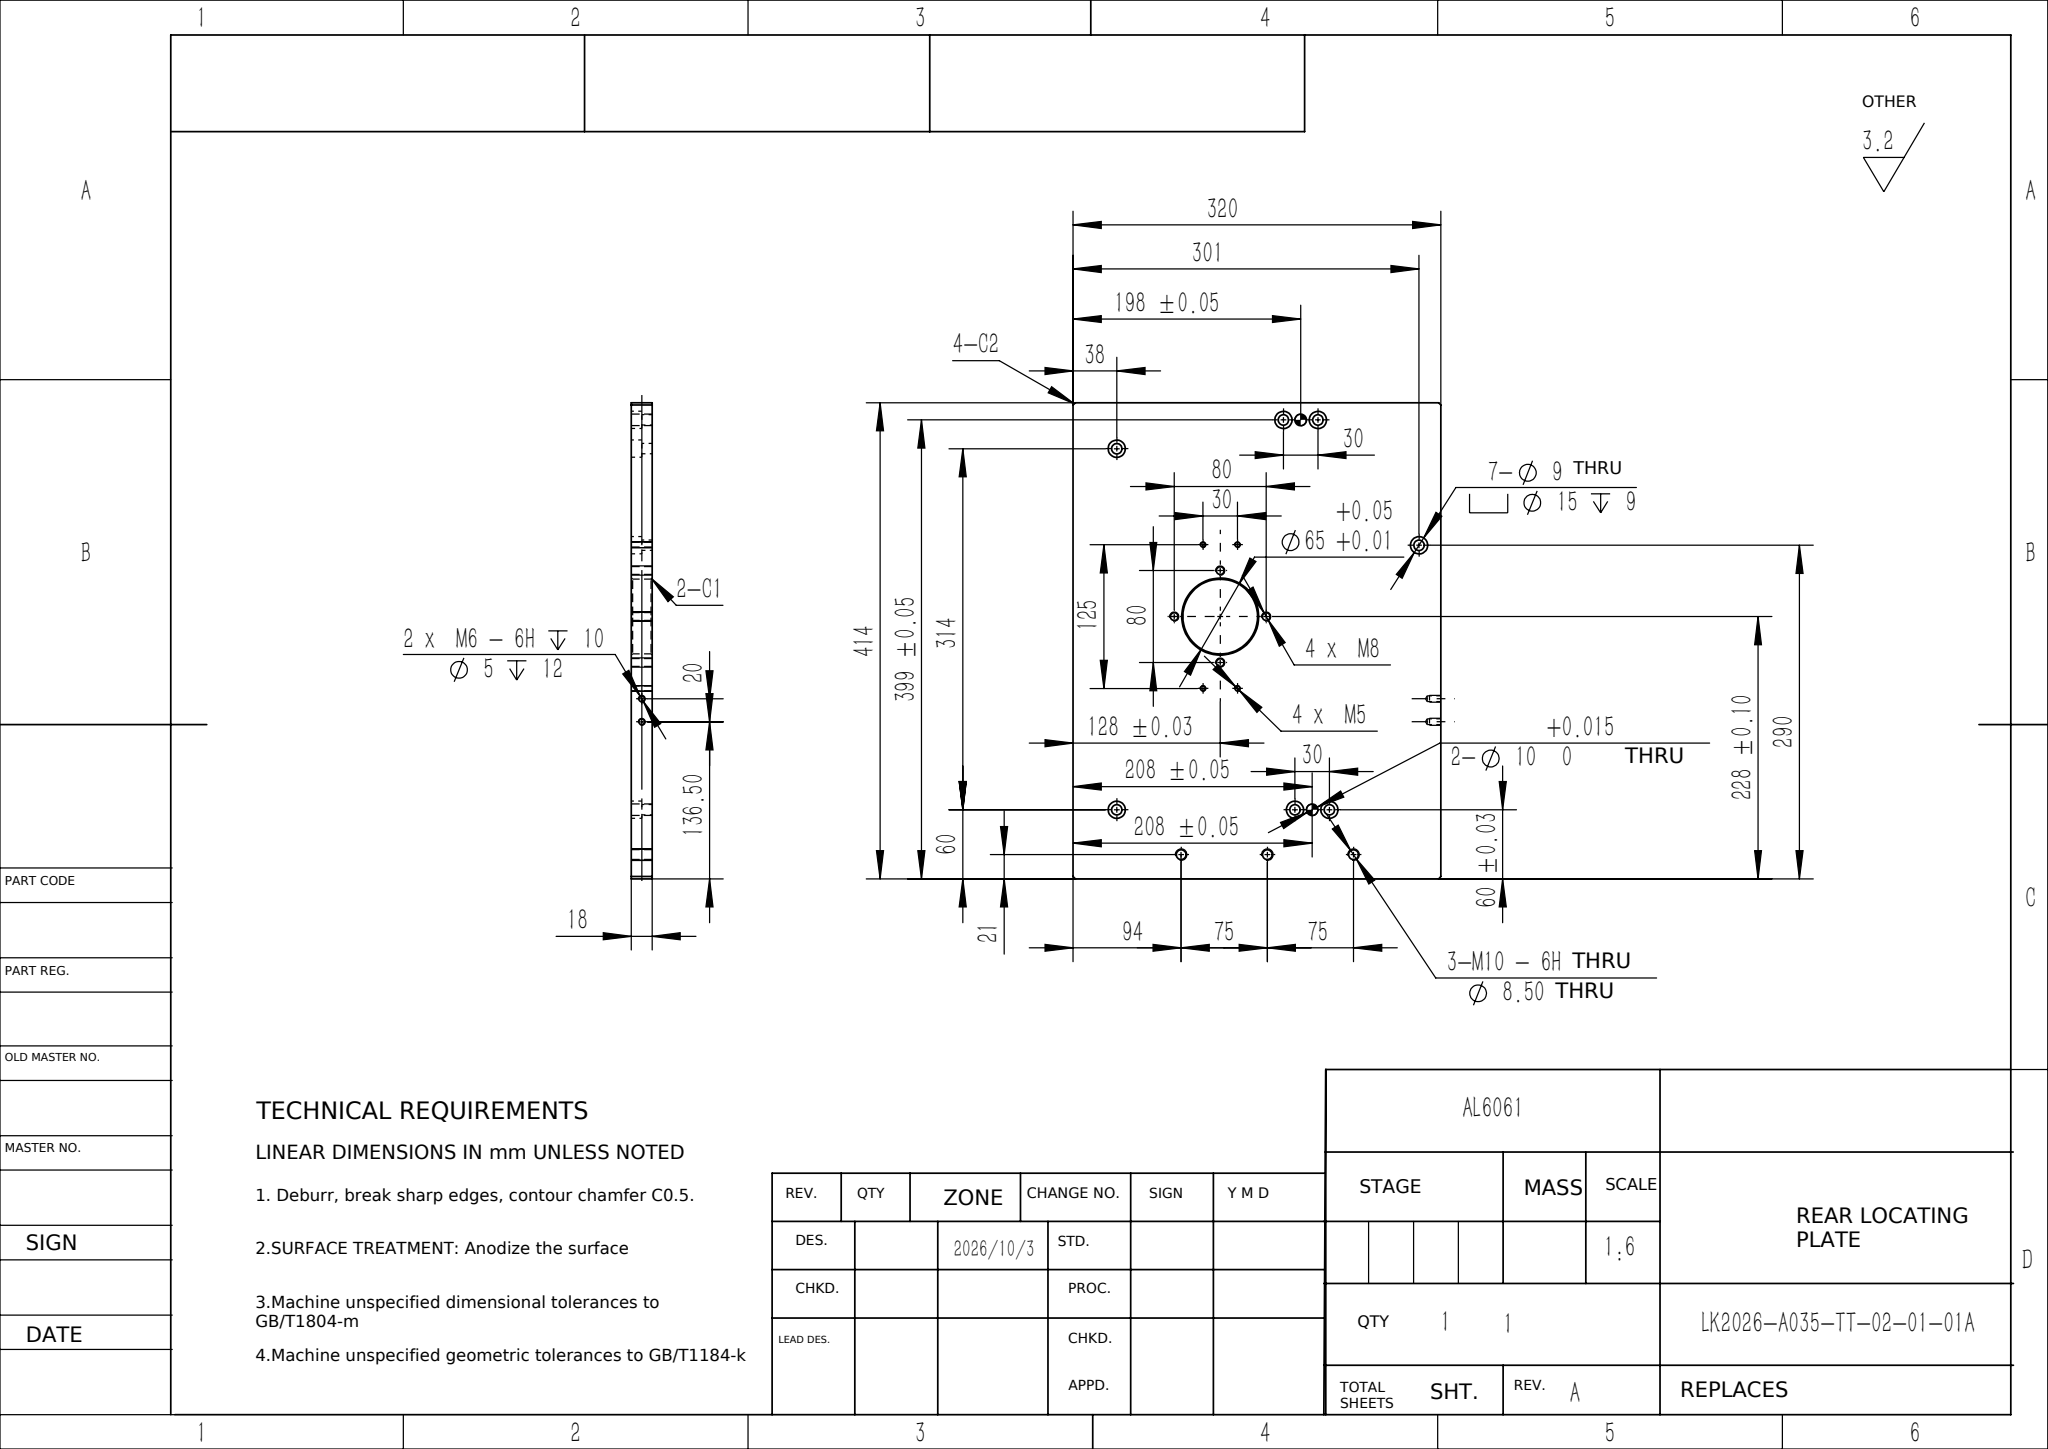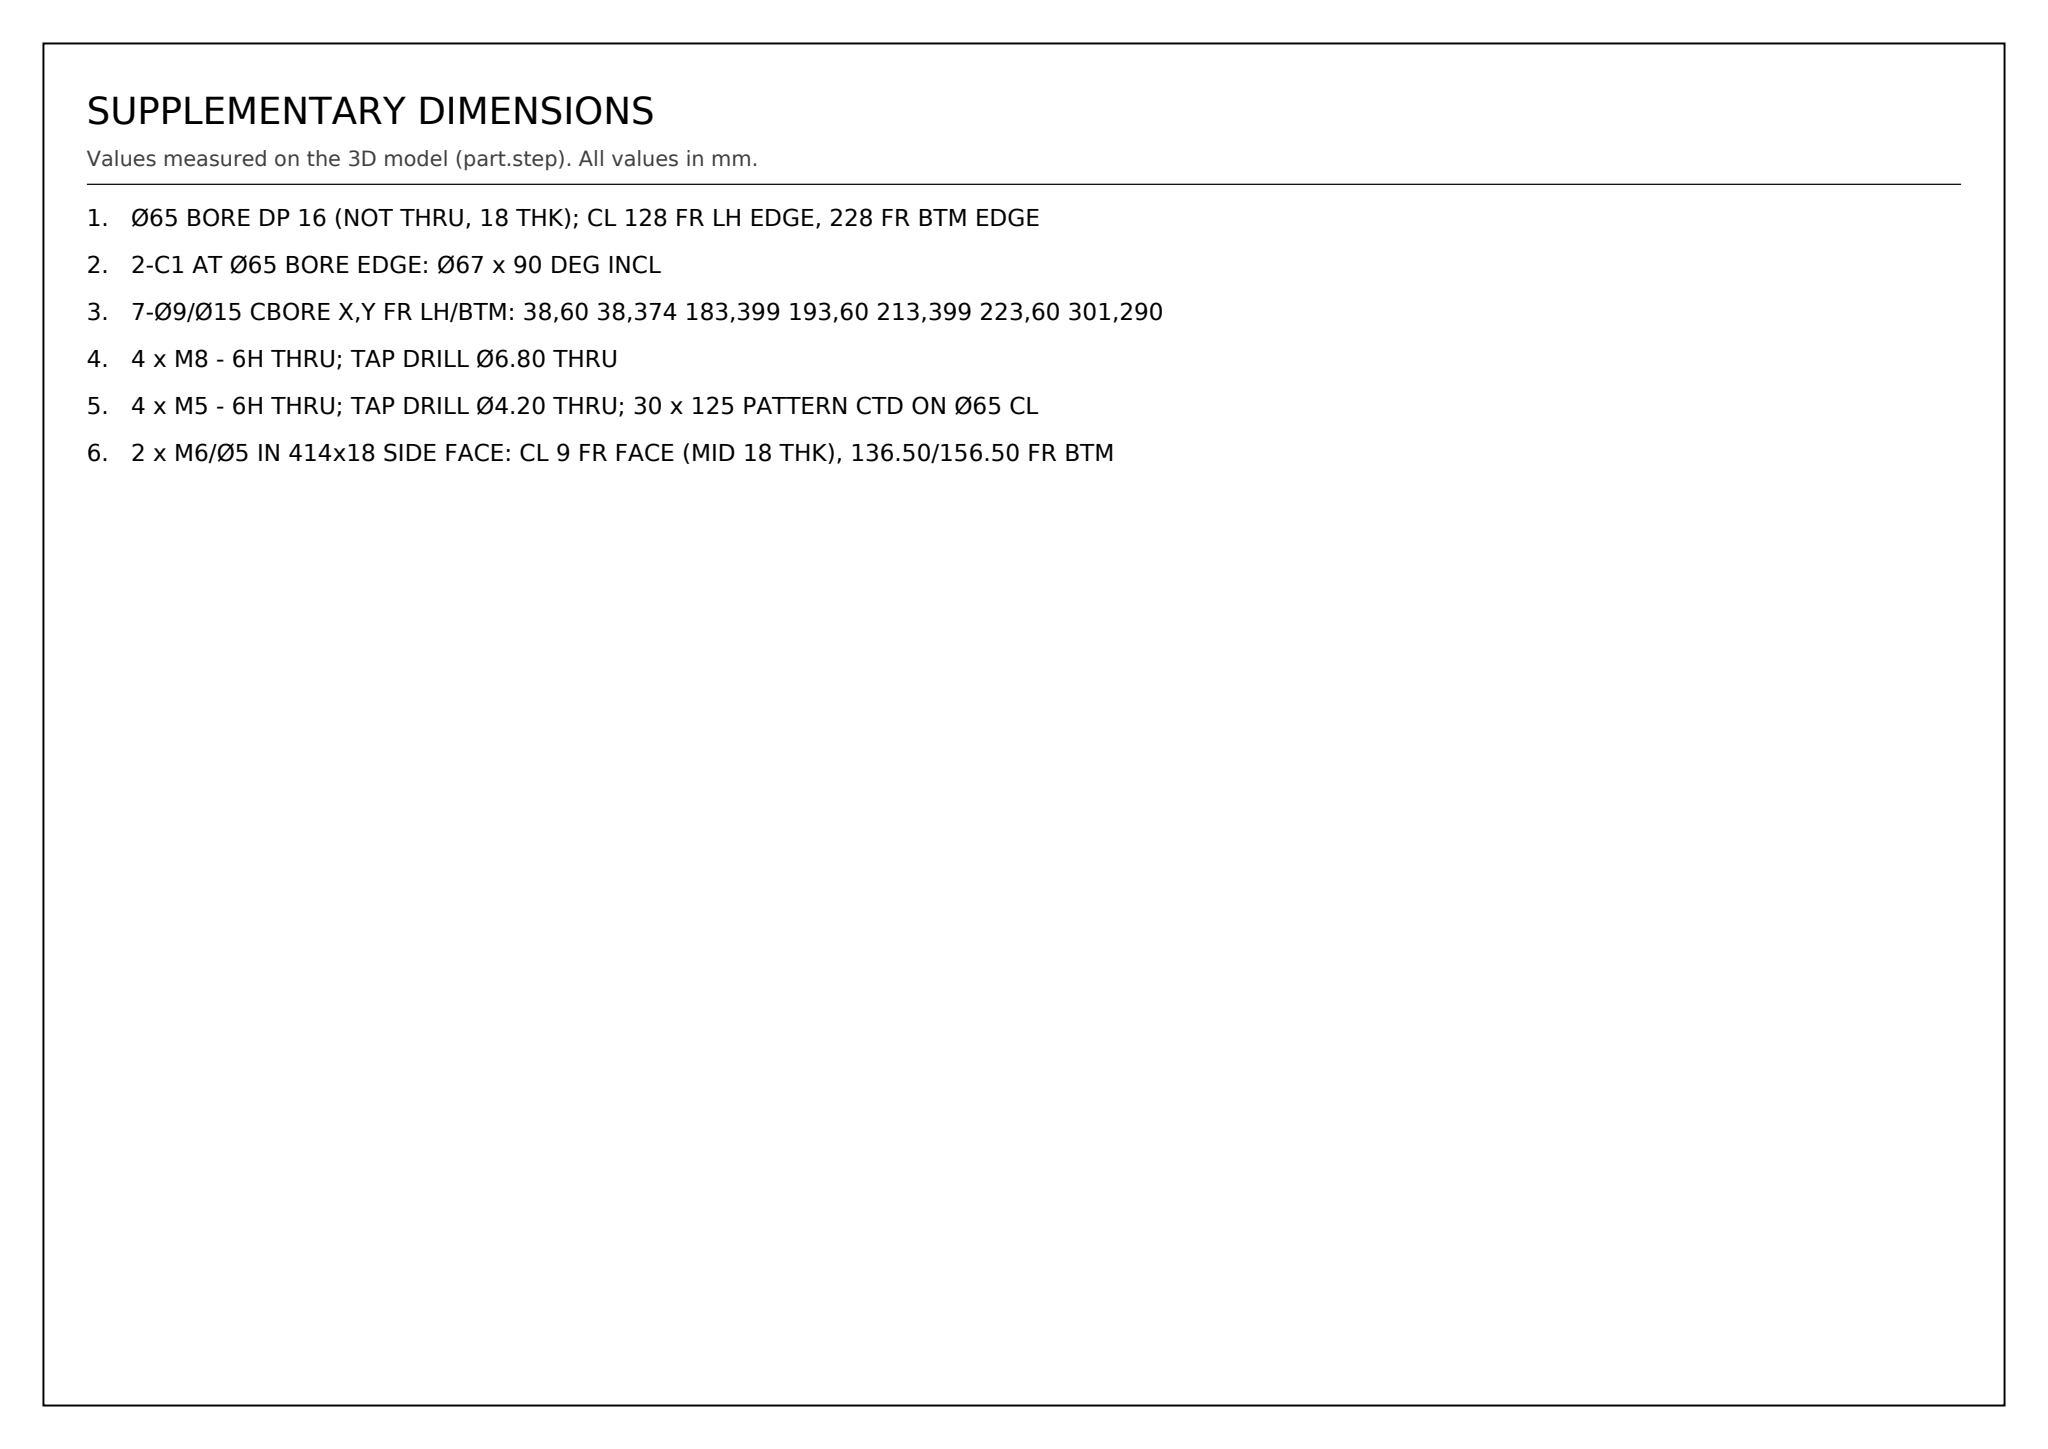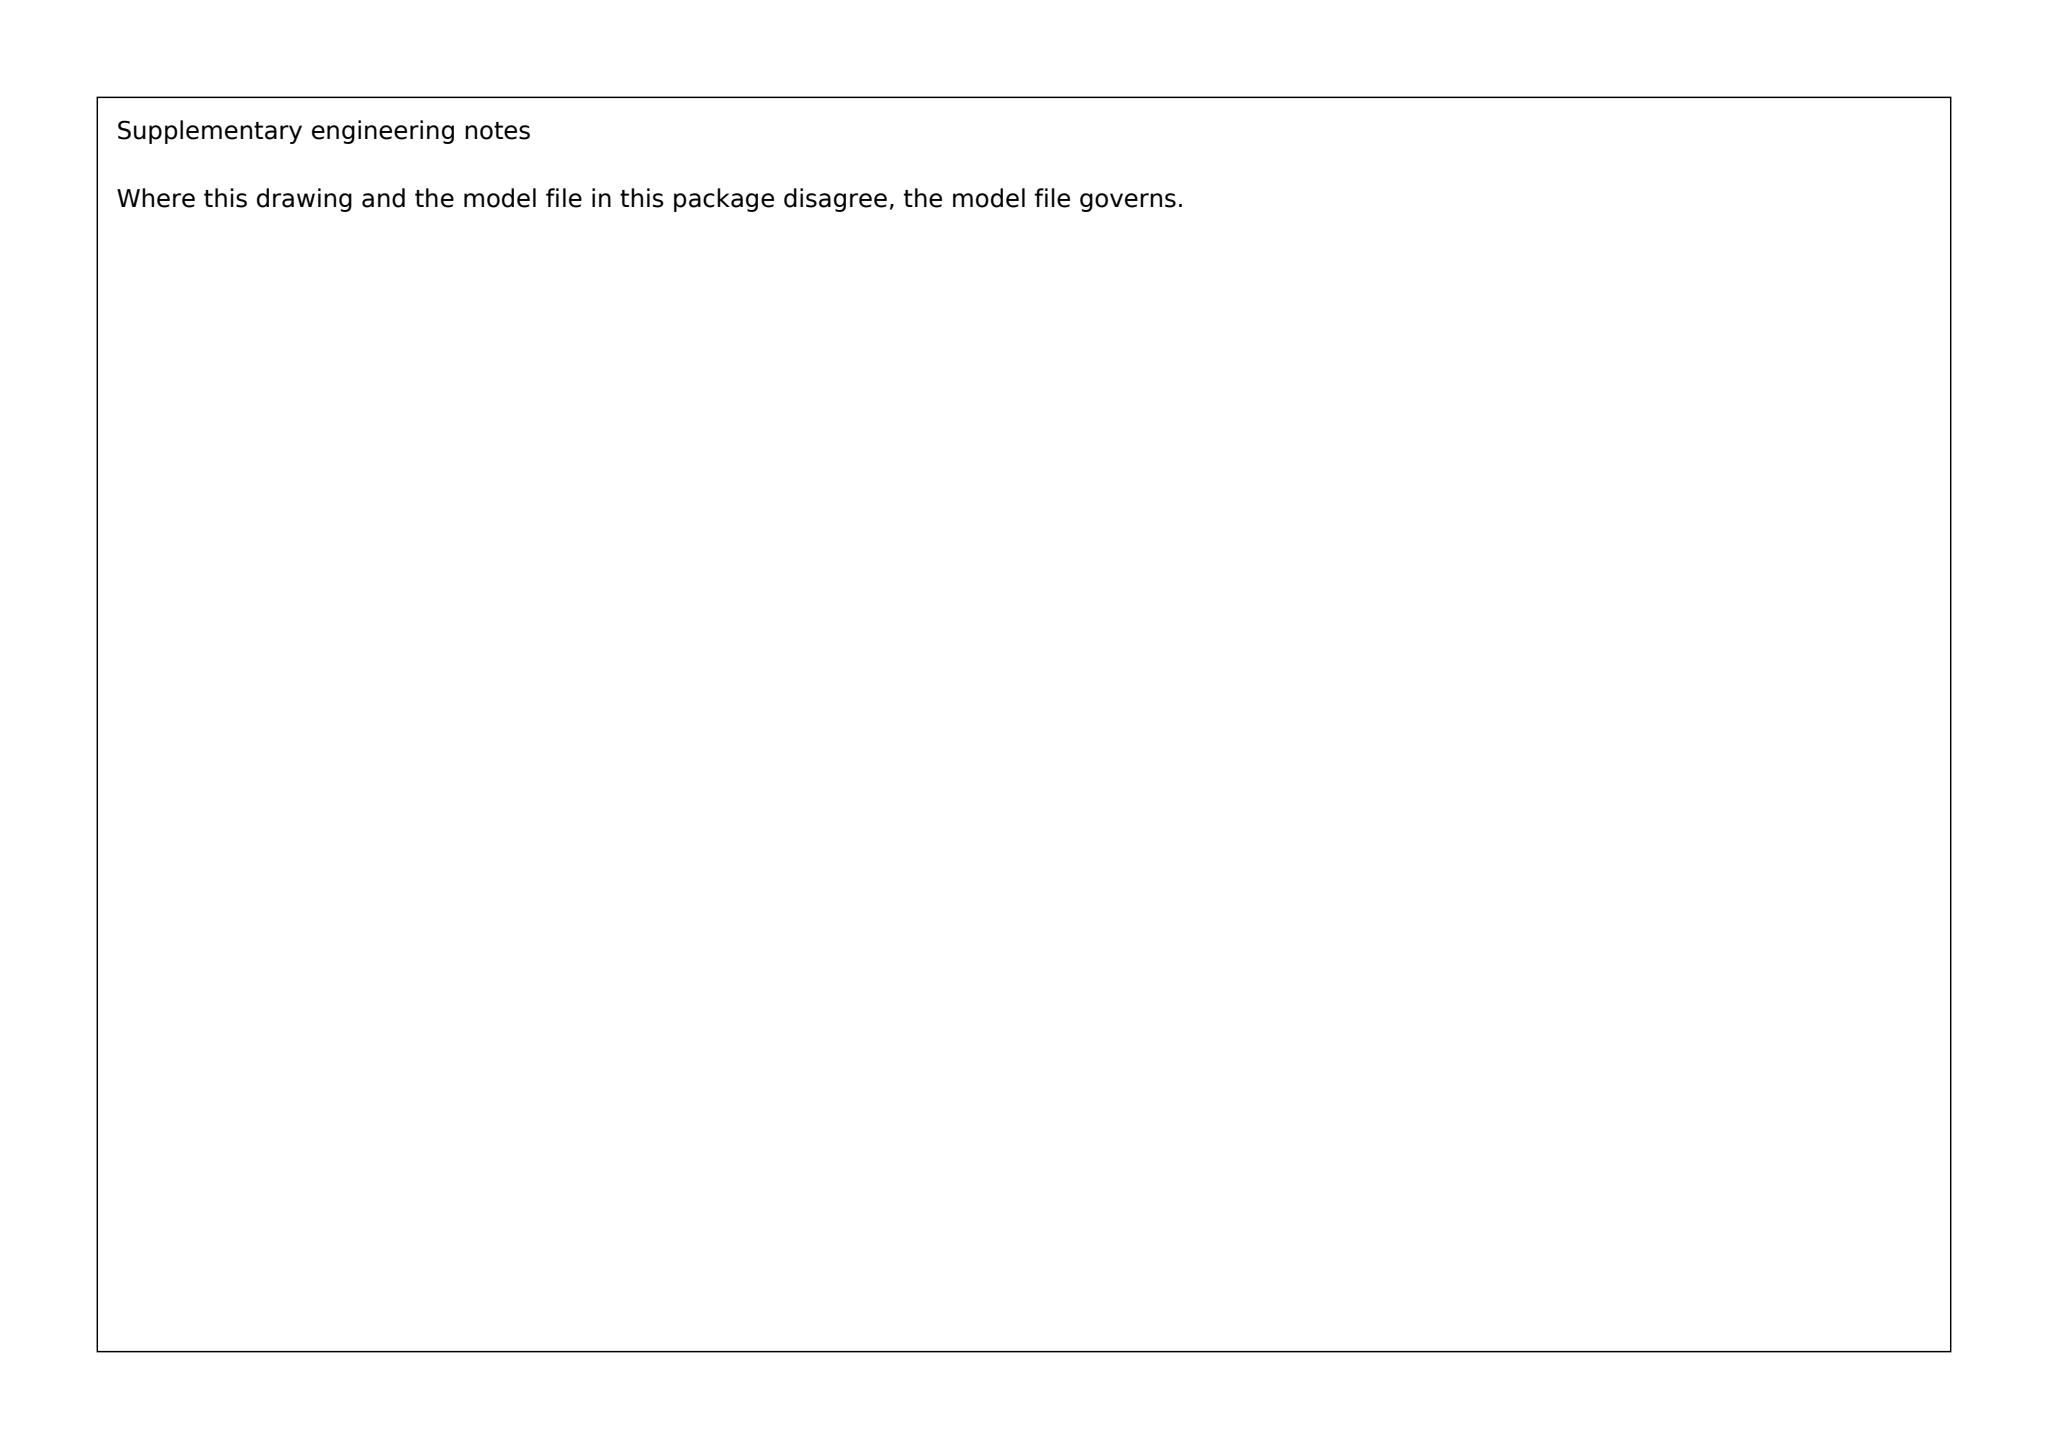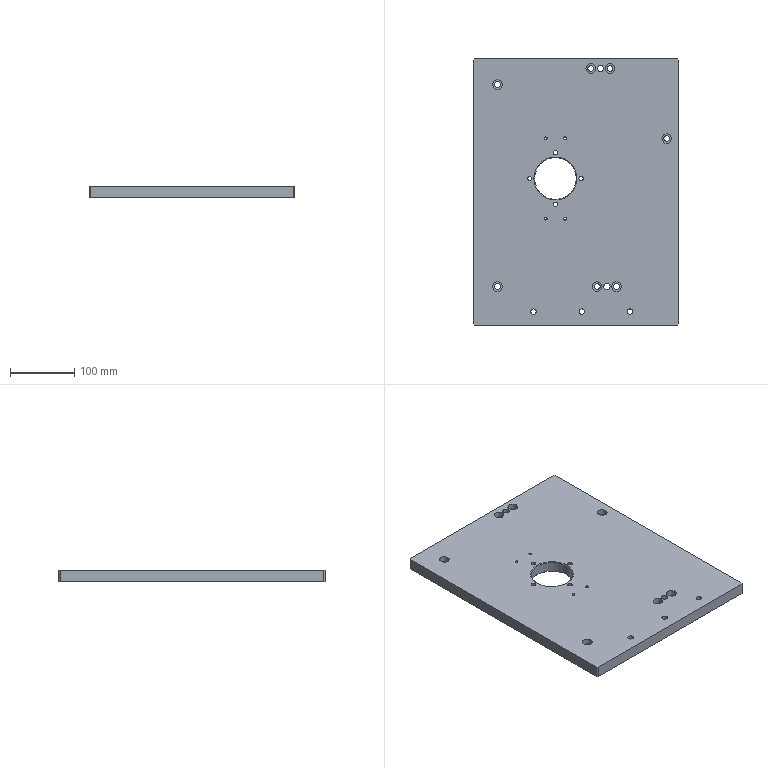Part | SolidWorks | mm | 1 solid | 85 faces | box 320 x 414 x 18 mm | volume 2299424 mm3 | cylinder 60 | plane 17 | cone 8 | commonest cylinder face diameters 15 x14 9 x14 4.2 x8 6.8 x8 8.5 x6 5 x4 10 x4 65 x2
Drawing notes:
Ø65 BORE DP 16 (NOT THRU, 18 THK); CL 128 FR LH EDGE, 228 FR BTM EDGE | from the solid: Ø65 z-axis cylinder at (128,228), length 16 < bbox z 18; bbox 320x414x18
2-C1 AT Ø65 BORE EDGE: Ø67 x 90 DEG INCL | from the solid: cones 90 deg included, ref dia 65 and 67, qty 2 at Ø65 bore
7-Ø9/Ø15 CBORE X,Y FR LH/BTM: 38,60 38,374 183,399 193,60 213,399 223,60 301,290 | from the solid: Ø9/Ø15 cbore axes (38,60),(38,374),(183,399),(193,60),(213,399),(223,60),(301,290)
4 x M8 - 6H THRU; TAP DRILL Ø6.80 THRU | from the solid: Ø6.8 z-axis cylinders at (88,228),(128,188),(128,268),(168,228), length 18 = full 18 thk
4 x M5 - 6H THRU; TAP DRILL Ø4.20 THRU; 30 x 125 PATTERN CTD ON Ø65 CL | from the solid: Ø4.2 cylinders at (113/143,165.5/290.5), L=18 thru; mid = (128,228) = bore CL
2 x M6/Ø5 IN 414x18 SIDE FACE: CL 9 FR FACE (MID 18 THK), 136.50/156.50 FR BTM | from the solid: Ø5 x-axis cylinders at z=9.0, y=136.5 & 156.5, length 12; bbox z 18
build123d program:
from build123d import *

# Parameters (mm, degrees)
SKETCH1_W                                         = 320
SKETCH1_H                                         = 414
BOSS_EXTRUDE1_DEPTH                               = 18
SKETCH8_R                                         = 32.5
CUT_EXTRUDE1_DEPTH                                = 263.246
HOLE_SIZE_ACCORDING_TO_HEXAGON_SOCKET_D           = 9
HOLE_SIZE_ACCORDING_TO_HEXAGON_SOCKET_CBORE_D     = 15
HOLE_SIZE_ACCORDING_TO_HEXAGON_SOCKET_CBORE_DEPTH = 9
M10_TAPPED_HOLE1_D                                = 8.5
SIZE_MM_DOWEL_PIN_HOLE_1_D                        = 10
M8_TAPPED_HOLE1_D                                 = 6.8
M6_TAPPED_HOLE2_D                                 = 5
M6_TAPPED_HOLE2_DEPTH                             = 12
M6_TAPPED_HOLE2_TIP                               = 1.502
CHAMFER1_SIZE                                     = 2
M5_TAPPED_HOLE1_D                                 = 4.2
CHAMFER2_SIZE                                     = 1


with BuildPart() as part:
    # Sketch1 → Boss-Extrude1 (new body)
    with BuildSketch(Plane.XY):
        Rectangle(SKETCH1_W, SKETCH1_H)
    extrude(amount=BOSS_EXTRUDE1_DEPTH)

    # Sketch8 → Cut-Extrude1 (cut, through all)
    with BuildSketch(Plane.XY.offset(18)):
        with Locations((-32, 21)):
            Circle(SKETCH8_R)
    extrude(amount=-CUT_EXTRUDE1_DEPTH, mode=Mode.SUBTRACT)

    # Hole Size _according to_ Hexagon Socket (through all)
    with Locations(Plane.XY.offset(18)):
        with Locations((-122, 167), (33, -147), (63, -147), (23, 192), (53, 192), (141, 83), (-122, -147)):
            CounterBoreHole(HOLE_SIZE_ACCORDING_TO_HEXAGON_SOCKET_D / 2, HOLE_SIZE_ACCORDING_TO_HEXAGON_SOCKET_CBORE_D / 2, HOLE_SIZE_ACCORDING_TO_HEXAGON_SOCKET_CBORE_DEPTH)

    # M10 Tapped Hole1 (through all)
    with Locations(Plane.XY.offset(18)):
        with Locations((84, -186), (9, -186), (-66, -186)):
            Hole(M10_TAPPED_HOLE1_D / 2)

    # Size mm Dowel Pin Hole 1 (through all)
    with Locations(Plane.XY.offset(18)):
        with Locations((38, 192), (48, -147)):
            Hole(SIZE_MM_DOWEL_PIN_HOLE_1_D / 2)

    # M8 Tapped Hole1 (through all)
    with Locations(Plane.XY.offset(18)):
        with Locations((-72, 21), (-32, 61), (8, 21), (-32, -19)):
            Hole(M8_TAPPED_HOLE1_D / 2)

    # M6 Tapped Hole2
    with Locations(Plane(origin=(160, 0, 0), x_dir=(0, 0, -1), z_dir=(1, 0, 0))):
        with Locations((-9, -50.5), (-9, -70.5)):
            Hole(M6_TAPPED_HOLE2_D / 2, depth=M6_TAPPED_HOLE2_DEPTH)
            with Locations((0, 0, -(M6_TAPPED_HOLE2_DEPTH + M6_TAPPED_HOLE2_TIP / 2))):  # 118° drill point
                Cone(0, M6_TAPPED_HOLE2_D / 2, M6_TAPPED_HOLE2_TIP, mode=Mode.SUBTRACT)

    # Chamfer1
    chamfer1_edges = [part.edges().sort_by_distance(p)[0] for p in [
        (160, -207, 9),
        (-160, -207, 9),
        (-160, 207, 9),
        (160, 207, 9),
    ]]
    chamfer(chamfer1_edges, length=CHAMFER1_SIZE)

    # M5 Tapped Hole1 (through all)
    with Locations(Plane.XY.offset(18)):
        with Locations((-17, -41.5), (-47, -41.5), (-47, 83.5), (-17, 83.5)):
            Hole(M5_TAPPED_HOLE1_D / 2)

    # Chamfer2
    chamfer2_edges = [part.edges().sort_by_distance(p)[0] for p in [
        (-64.5, 21, 0),
        (-64.5, 21, 18),
    ]]
    chamfer(chamfer2_edges, length=CHAMFER2_SIZE)


solid = part.part